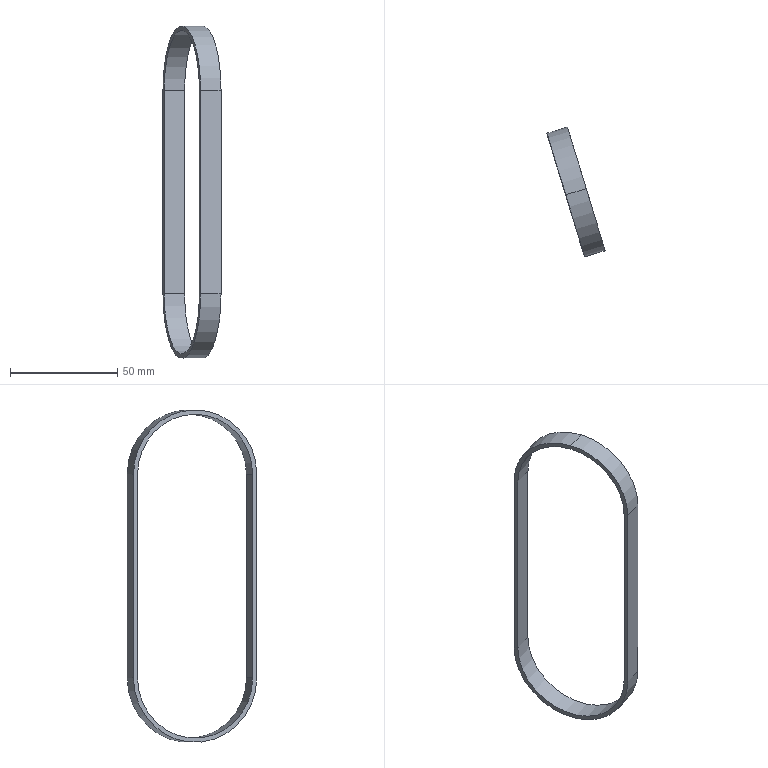Component | SolidWorks | v1_Part1-2112091-1 | 1 solid | 12 faces | box 27.13 x 60.5 x 155.2 mm | volume 7457 mm3 | cylinder 6 | plane 6 | commonest cylinder face diameters 56.2 x3 60.2 x3
build123d program:
from build123d import *

# Parameters (mm, degrees)
EXTRUDE_THIN1_DEPTH = 10


with BuildPart() as part:
    # Sketch1 → Extrude-Thin1 (new body)
    with BuildSketch(Plane.XY):
        with BuildLine():
            Line((95, -30.1), (0, -30.1))
            ThreePointArc((0, -30.1), (-30.1, 0), (0, 30.1))
            Line((0, 30.1), (95, 30.1))
            ThreePointArc((95, 30.1), (125.1, 0), (95, -30.1))
        make_face()
        with BuildLine():
            Line((95, -28.1), (0, -28.1))
            ThreePointArc((0, -28.1), (-28.1, 0), (0, 28.1))
            Line((0, 28.1), (95, 28.1))
            ThreePointArc((95, 28.1), (123.1, 0), (95, -28.1))
        make_face(mode=Mode.SUBTRACT)
    extrude(amount=EXTRUDE_THIN1_DEPTH)


solid = part.part

# Placed as in the assembly
solid = solid.moved(Location((193.934, -227.048, 280.239), (-90, 73.032, -90)))
STEP:
#1=COLOUR_RGB('',0.7922,0.8196,0.9333);
#2=FILL_AREA_STYLE_COLOUR('',#1);
#3=FILL_AREA_STYLE('',(#2));
#4=SURFACE_STYLE_FILL_AREA(#3);
#5=SURFACE_SIDE_STYLE('',(#4));
#6=SURFACE_STYLE_USAGE(.BOTH.,#5);
#7=PRESENTATION_STYLE_ASSIGNMENT((#6));
#8=CARTESIAN_POINT('',(7.689,-7.766,14.773));
#9=VERTEX_POINT('',#8);
#10=CARTESIAN_POINT('',(8.012,-8.824,15.879));
#11=VERTEX_POINT('',#10);
#12=CARTESIAN_POINT('',(8.012,-8.824,14.773));
#13=DIRECTION('',(0.9565,0.2918,0.));
#14=DIRECTION('',(0.,0.,-1.));
#15=AXIS2_PLACEMENT_3D('',#12,#13,#14);
#16=CIRCLE('',#15,1.106);
#17=EDGE_CURVE('',#9,#11,#16,.T.);
#18=ORIENTED_EDGE('',*,*,#17,.T.);
#19=CARTESIAN_POINT('',(7.635,-8.939,15.879));
#20=VERTEX_POINT('',#19);
#21=CARTESIAN_POINT('',(8.012,-8.824,15.879));
#22=DIRECTION('',(-0.9565,-0.2918,-0.));
#23=VECTOR('',#22,39.37);
#24=LINE('',#21,#23);
#25=EDGE_CURVE('',#11,#20,#24,.T.);
#26=ORIENTED_EDGE('',*,*,#25,.T.);
#27=CARTESIAN_POINT('',(7.312,-7.881,14.773));
#28=VERTEX_POINT('',#27);
#29=CARTESIAN_POINT('',(7.635,-8.939,14.773));
#30=DIRECTION('',(0.9565,0.2918,0.));
#31=DIRECTION('',(0.,0.,-1.));
#32=AXIS2_PLACEMENT_3D('',#29,#30,#31);
#33=CIRCLE('',#32,1.106);
#34=EDGE_CURVE('',#28,#20,#33,.T.);
#35=ORIENTED_EDGE('',*,*,#34,.F.);
#36=CARTESIAN_POINT('',(7.689,-7.766,14.773));
#37=DIRECTION('',(-0.9565,-0.2918,-0.));
#38=VECTOR('',#37,39.37);
#39=LINE('',#36,#38);
#40=EDGE_CURVE('',#9,#28,#39,.T.);
#41=ORIENTED_EDGE('',*,*,#40,.F.);
#42=EDGE_LOOP('',(#18,#26,#35,#41));
#43=FACE_OUTER_BOUND('',#42,.T.);
#44=CARTESIAN_POINT('',(8.012,-8.824,14.773));
#45=DIRECTION('',(-0.9565,-0.2918,-0.));
#46=DIRECTION('',(-0.,-0.,1.));
#47=AXIS2_PLACEMENT_3D('',#44,#45,#46);
#48=CYLINDRICAL_SURFACE('',#47,1.106);
#49=ADVANCED_FACE('',(#43),#48,.F.);
#50=CARTESIAN_POINT('',(8.012,-8.824,15.958));
#51=VERTEX_POINT('',#50);
#52=CARTESIAN_POINT('',(8.358,-9.957,14.773));
#53=VERTEX_POINT('',#52);
#54=CARTESIAN_POINT('',(8.012,-8.824,14.773));
#55=DIRECTION('',(0.9565,0.2918,0.));
#56=DIRECTION('',(0.,0.,-1.));
#57=AXIS2_PLACEMENT_3D('',#54,#55,#56);
#58=CIRCLE('',#57,1.185);
#59=EDGE_CURVE('',#51,#53,#58,.T.);
#60=ORIENTED_EDGE('',*,*,#59,.F.);
#61=CARTESIAN_POINT('',(7.635,-8.939,15.958));
#62=VERTEX_POINT('',#61);
#63=CARTESIAN_POINT('',(8.012,-8.824,15.958));
#64=DIRECTION('',(-0.9565,-0.2918,-0.));
#65=VECTOR('',#64,39.37);
#66=LINE('',#63,#65);
#67=EDGE_CURVE('',#51,#62,#66,.T.);
#68=ORIENTED_EDGE('',*,*,#67,.T.);
#69=CARTESIAN_POINT('',(7.981,-10.072,14.773));
#70=VERTEX_POINT('',#69);
#71=CARTESIAN_POINT('',(7.635,-8.939,14.773));
#72=DIRECTION('',(0.9565,0.2918,0.));
#73=DIRECTION('',(0.,0.,-1.));
#74=AXIS2_PLACEMENT_3D('',#71,#72,#73);
#75=CIRCLE('',#74,1.185);
#76=EDGE_CURVE('',#62,#70,#75,.T.);
#77=ORIENTED_EDGE('',*,*,#76,.T.);
#78=CARTESIAN_POINT('',(8.358,-9.957,14.773));
#79=DIRECTION('',(-0.9565,-0.2918,-0.));
#80=VECTOR('',#79,39.37);
#81=LINE('',#78,#80);
#82=EDGE_CURVE('',#53,#70,#81,.T.);
#83=ORIENTED_EDGE('',*,*,#82,.F.);
#84=EDGE_LOOP('',(#60,#68,#77,#83));
#85=FACE_OUTER_BOUND('',#84,.T.);
#86=CARTESIAN_POINT('',(8.012,-8.824,14.773));
#87=DIRECTION('',(-0.9565,-0.2918,-0.));
#88=DIRECTION('',(-0.,-0.,1.));
#89=AXIS2_PLACEMENT_3D('',#86,#87,#88);
#90=CYLINDRICAL_SURFACE('',#89,1.185);
#91=ADVANCED_FACE('',(#85),#90,.T.);
#92=CARTESIAN_POINT('',(8.358,-9.957,11.033));
#93=VERTEX_POINT('',#92);
#94=CARTESIAN_POINT('',(7.666,-7.691,11.033));
#95=VERTEX_POINT('',#94);
#96=CARTESIAN_POINT('',(8.012,-8.824,11.033));
#97=DIRECTION('',(0.9565,0.2918,0.));
#98=DIRECTION('',(0.,0.,-1.));
#99=AXIS2_PLACEMENT_3D('',#96,#97,#98);
#100=CIRCLE('',#99,1.185);
#101=EDGE_CURVE('',#93,#95,#100,.T.);
#102=ORIENTED_EDGE('',*,*,#101,.T.);
#103=CARTESIAN_POINT('',(7.666,-7.691,14.773));
#104=VERTEX_POINT('',#103);
#105=CARTESIAN_POINT('',(7.666,-7.691,14.773));
#106=DIRECTION('',(-0.,-0.,1.));
#107=VECTOR('',#106,39.37);
#108=LINE('',#105,#107);
#109=EDGE_CURVE('',#95,#104,#108,.T.);
#110=ORIENTED_EDGE('',*,*,#109,.T.);
#111=CARTESIAN_POINT('',(8.012,-8.824,14.773));
#112=DIRECTION('',(0.9565,0.2918,0.));
#113=DIRECTION('',(0.,0.,-1.));
#114=AXIS2_PLACEMENT_3D('',#111,#112,#113);
#115=CIRCLE('',#114,1.185);
#116=EDGE_CURVE('',#104,#51,#115,.T.);
#117=ORIENTED_EDGE('',*,*,#116,.T.);
#118=ORIENTED_EDGE('',*,*,#59,.T.);
#119=CARTESIAN_POINT('',(8.358,-9.957,11.033));
#120=DIRECTION('',(0.,0.,-1.));
#121=VECTOR('',#120,39.37);
#122=LINE('',#119,#121);
#123=EDGE_CURVE('',#53,#93,#122,.T.);
#124=ORIENTED_EDGE('',*,*,#123,.T.);
#125=EDGE_LOOP('',(#102,#110,#117,#118,#124));
#126=FACE_OUTER_BOUND('',#125,.T.);
#127=CARTESIAN_POINT('',(7.689,-7.766,11.033));
#128=VERTEX_POINT('',#127);
#129=CARTESIAN_POINT('',(7.689,-7.766,14.773));
#130=DIRECTION('',(-0.,-0.,1.));
#131=VECTOR('',#130,39.37);
#132=LINE('',#129,#131);
#133=EDGE_CURVE('',#128,#9,#132,.T.);
#134=ORIENTED_EDGE('',*,*,#133,.F.);
#135=CARTESIAN_POINT('',(8.335,-9.882,11.033));
#136=VERTEX_POINT('',#135);
#137=CARTESIAN_POINT('',(8.012,-8.824,11.033));
#138=DIRECTION('',(0.9565,0.2918,0.));
#139=DIRECTION('',(0.,0.,-1.));
#140=AXIS2_PLACEMENT_3D('',#137,#138,#139);
#141=CIRCLE('',#140,1.106);
#142=EDGE_CURVE('',#136,#128,#141,.T.);
#143=ORIENTED_EDGE('',*,*,#142,.F.);
#144=CARTESIAN_POINT('',(8.335,-9.882,14.773));
#145=VERTEX_POINT('',#144);
#146=CARTESIAN_POINT('',(8.335,-9.882,11.033));
#147=DIRECTION('',(0.,0.,-1.));
#148=VECTOR('',#147,39.37);
#149=LINE('',#146,#148);
#150=EDGE_CURVE('',#145,#136,#149,.T.);
#151=ORIENTED_EDGE('',*,*,#150,.F.);
#152=CARTESIAN_POINT('',(8.012,-8.824,14.773));
#153=DIRECTION('',(0.9565,0.2918,0.));
#154=DIRECTION('',(0.,0.,-1.));
#155=AXIS2_PLACEMENT_3D('',#152,#153,#154);
#156=CIRCLE('',#155,1.106);
#157=EDGE_CURVE('',#11,#145,#156,.T.);
#158=ORIENTED_EDGE('',*,*,#157,.F.);
#159=ORIENTED_EDGE('',*,*,#17,.F.);
#160=EDGE_LOOP('',(#134,#143,#151,#158,#159));
#161=FACE_BOUND('',#160,.T.);
#162=CARTESIAN_POINT('',(8.012,-8.824,11.033));
#163=DIRECTION('',(0.9565,0.2918,0.));
#164=DIRECTION('',(0.,0.,-1.));
#165=AXIS2_PLACEMENT_3D('',#162,#163,#164);
#166=PLANE('',#165);
#167=ADVANCED_FACE('',(#126,#161),#166,.T.);
#168=CARTESIAN_POINT('',(7.981,-10.072,11.033));
#169=VERTEX_POINT('',#168);
#170=CARTESIAN_POINT('',(7.289,-7.805,11.033));
#171=VERTEX_POINT('',#170);
#172=CARTESIAN_POINT('',(7.635,-8.939,11.033));
#173=DIRECTION('',(0.9565,0.2918,0.));
#174=DIRECTION('',(0.,0.,-1.));
#175=AXIS2_PLACEMENT_3D('',#172,#173,#174);
#176=CIRCLE('',#175,1.185);
#177=EDGE_CURVE('',#169,#171,#176,.T.);
#178=ORIENTED_EDGE('',*,*,#177,.F.);
#179=CARTESIAN_POINT('',(7.981,-10.072,11.033));
#180=DIRECTION('',(0.,0.,-1.));
#181=VECTOR('',#180,39.37);
#182=LINE('',#179,#181);
#183=EDGE_CURVE('',#70,#169,#182,.T.);
#184=ORIENTED_EDGE('',*,*,#183,.F.);
#185=ORIENTED_EDGE('',*,*,#76,.F.);
#186=CARTESIAN_POINT('',(7.289,-7.805,14.773));
#187=VERTEX_POINT('',#186);
#188=CARTESIAN_POINT('',(7.635,-8.939,14.773));
#189=DIRECTION('',(0.9565,0.2918,0.));
#190=DIRECTION('',(0.,0.,-1.));
#191=AXIS2_PLACEMENT_3D('',#188,#189,#190);
#192=CIRCLE('',#191,1.185);
#193=EDGE_CURVE('',#187,#62,#192,.T.);
#194=ORIENTED_EDGE('',*,*,#193,.F.);
#195=CARTESIAN_POINT('',(7.289,-7.805,14.773));
#196=DIRECTION('',(-0.,-0.,1.));
#197=VECTOR('',#196,39.37);
#198=LINE('',#195,#197);
#199=EDGE_CURVE('',#171,#187,#198,.T.);
#200=ORIENTED_EDGE('',*,*,#199,.F.);
#201=EDGE_LOOP('',(#178,#184,#185,#194,#200));
#202=FACE_OUTER_BOUND('',#201,.T.);
#203=CARTESIAN_POINT('',(7.958,-9.997,11.033));
#204=VERTEX_POINT('',#203);
#205=CARTESIAN_POINT('',(7.312,-7.881,11.033));
#206=VERTEX_POINT('',#205);
#207=CARTESIAN_POINT('',(7.635,-8.939,11.033));
#208=DIRECTION('',(0.9565,0.2918,0.));
#209=DIRECTION('',(0.,0.,-1.));
#210=AXIS2_PLACEMENT_3D('',#207,#208,#209);
#211=CIRCLE('',#210,1.106);
#212=EDGE_CURVE('',#204,#206,#211,.T.);
#213=ORIENTED_EDGE('',*,*,#212,.T.);
#214=CARTESIAN_POINT('',(7.312,-7.881,14.773));
#215=DIRECTION('',(-0.,-0.,1.));
#216=VECTOR('',#215,39.37);
#217=LINE('',#214,#216);
#218=EDGE_CURVE('',#206,#28,#217,.T.);
#219=ORIENTED_EDGE('',*,*,#218,.T.);
#220=ORIENTED_EDGE('',*,*,#34,.T.);
#221=CARTESIAN_POINT('',(7.958,-9.997,14.773));
#222=VERTEX_POINT('',#221);
#223=CARTESIAN_POINT('',(7.635,-8.939,14.773));
#224=DIRECTION('',(0.9565,0.2918,0.));
#225=DIRECTION('',(0.,0.,-1.));
#226=AXIS2_PLACEMENT_3D('',#223,#224,#225);
#227=CIRCLE('',#226,1.106);
#228=EDGE_CURVE('',#20,#222,#227,.T.);
#229=ORIENTED_EDGE('',*,*,#228,.T.);
#230=CARTESIAN_POINT('',(7.958,-9.997,11.033));
#231=DIRECTION('',(0.,0.,-1.));
#232=VECTOR('',#231,39.37);
#233=LINE('',#230,#232);
#234=EDGE_CURVE('',#222,#204,#233,.T.);
#235=ORIENTED_EDGE('',*,*,#234,.T.);
#236=EDGE_LOOP('',(#213,#219,#220,#229,#235));
#237=FACE_BOUND('',#236,.T.);
#238=CARTESIAN_POINT('',(7.635,-8.939,11.033));
#239=DIRECTION('',(0.9565,0.2918,0.));
#240=DIRECTION('',(0.,0.,-1.));
#241=AXIS2_PLACEMENT_3D('',#238,#239,#240);
#242=PLANE('',#241);
#243=ADVANCED_FACE('',(#202,#237),#242,.F.);
#244=ORIENTED_EDGE('',*,*,#177,.T.);
#245=CARTESIAN_POINT('',(7.666,-7.691,11.033));
#246=DIRECTION('',(-0.9565,-0.2918,-0.));
#247=VECTOR('',#246,39.37);
#248=LINE('',#245,#247);
#249=EDGE_CURVE('',#95,#171,#248,.T.);
#250=ORIENTED_EDGE('',*,*,#249,.F.);
#251=ORIENTED_EDGE('',*,*,#101,.F.);
#252=CARTESIAN_POINT('',(8.358,-9.957,11.033));
#253=DIRECTION('',(-0.9565,-0.2918,-0.));
#254=VECTOR('',#253,39.37);
#255=LINE('',#252,#254);
#256=EDGE_CURVE('',#93,#169,#255,.T.);
#257=ORIENTED_EDGE('',*,*,#256,.T.);
#258=EDGE_LOOP('',(#244,#250,#251,#257));
#259=FACE_OUTER_BOUND('',#258,.T.);
#260=CARTESIAN_POINT('',(8.012,-8.824,11.033));
#261=DIRECTION('',(-0.9565,-0.2918,-0.));
#262=DIRECTION('',(-0.,-0.,1.));
#263=AXIS2_PLACEMENT_3D('',#260,#261,#262);
#264=CYLINDRICAL_SURFACE('',#263,1.185);
#265=ADVANCED_FACE('',(#259),#264,.T.);
#266=ORIENTED_EDGE('',*,*,#199,.T.);
#267=CARTESIAN_POINT('',(7.666,-7.691,14.773));
#268=DIRECTION('',(-0.9565,-0.2918,-0.));
#269=VECTOR('',#268,39.37);
#270=LINE('',#267,#269);
#271=EDGE_CURVE('',#104,#187,#270,.T.);
#272=ORIENTED_EDGE('',*,*,#271,.F.);
#273=ORIENTED_EDGE('',*,*,#109,.F.);
#274=ORIENTED_EDGE('',*,*,#249,.T.);
#275=EDGE_LOOP('',(#266,#272,#273,#274));
#276=FACE_OUTER_BOUND('',#275,.T.);
#277=CARTESIAN_POINT('',(7.666,-7.691,14.773));
#278=DIRECTION('',(0.2918,-0.9565,-0.));
#279=DIRECTION('',(-0.9565,-0.2918,-0.));
#280=AXIS2_PLACEMENT_3D('',#277,#278,#279);
#281=PLANE('',#280);
#282=ADVANCED_FACE('',(#276),#281,.F.);
#283=ORIENTED_EDGE('',*,*,#67,.F.);
#284=ORIENTED_EDGE('',*,*,#116,.F.);
#285=ORIENTED_EDGE('',*,*,#271,.T.);
#286=ORIENTED_EDGE('',*,*,#193,.T.);
#287=EDGE_LOOP('',(#283,#284,#285,#286));
#288=FACE_OUTER_BOUND('',#287,.T.);
#289=CARTESIAN_POINT('',(8.012,-8.824,14.773));
#290=DIRECTION('',(-0.9565,-0.2918,-0.));
#291=DIRECTION('',(-0.,-0.,1.));
#292=AXIS2_PLACEMENT_3D('',#289,#290,#291);
#293=CYLINDRICAL_SURFACE('',#292,1.185);
#294=ADVANCED_FACE('',(#288),#293,.T.);
#295=ORIENTED_EDGE('',*,*,#183,.T.);
#296=ORIENTED_EDGE('',*,*,#256,.F.);
#297=ORIENTED_EDGE('',*,*,#123,.F.);
#298=ORIENTED_EDGE('',*,*,#82,.T.);
#299=EDGE_LOOP('',(#295,#296,#297,#298));
#300=FACE_OUTER_BOUND('',#299,.T.);
#301=CARTESIAN_POINT('',(8.358,-9.957,11.033));
#302=DIRECTION('',(-0.2918,0.9565,0.));
#303=DIRECTION('',(0.9565,0.2918,0.));
#304=AXIS2_PLACEMENT_3D('',#301,#302,#303);
#305=PLANE('',#304);
#306=ADVANCED_FACE('',(#300),#305,.F.);
#307=ORIENTED_EDGE('',*,*,#212,.F.);
#308=CARTESIAN_POINT('',(8.335,-9.882,11.033));
#309=DIRECTION('',(-0.9565,-0.2918,-0.));
#310=VECTOR('',#309,39.37);
#311=LINE('',#308,#310);
#312=EDGE_CURVE('',#136,#204,#311,.T.);
#313=ORIENTED_EDGE('',*,*,#312,.F.);
#314=ORIENTED_EDGE('',*,*,#142,.T.);
#315=CARTESIAN_POINT('',(7.689,-7.766,11.033));
#316=DIRECTION('',(-0.9565,-0.2918,-0.));
#317=VECTOR('',#316,39.37);
#318=LINE('',#315,#317);
#319=EDGE_CURVE('',#128,#206,#318,.T.);
#320=ORIENTED_EDGE('',*,*,#319,.T.);
#321=EDGE_LOOP('',(#307,#313,#314,#320));
#322=FACE_OUTER_BOUND('',#321,.T.);
#323=CARTESIAN_POINT('',(8.012,-8.824,11.033));
#324=DIRECTION('',(-0.9565,-0.2918,-0.));
#325=DIRECTION('',(-0.,-0.,1.));
#326=AXIS2_PLACEMENT_3D('',#323,#324,#325);
#327=CYLINDRICAL_SURFACE('',#326,1.106);
#328=ADVANCED_FACE('',(#322),#327,.F.);
#329=ORIENTED_EDGE('',*,*,#218,.F.);
#330=ORIENTED_EDGE('',*,*,#319,.F.);
#331=ORIENTED_EDGE('',*,*,#133,.T.);
#332=ORIENTED_EDGE('',*,*,#40,.T.);
#333=EDGE_LOOP('',(#329,#330,#331,#332));
#334=FACE_OUTER_BOUND('',#333,.T.);
#335=CARTESIAN_POINT('',(7.689,-7.766,14.773));
#336=DIRECTION('',(0.2918,-0.9565,-0.));
#337=DIRECTION('',(-0.9565,-0.2918,-0.));
#338=AXIS2_PLACEMENT_3D('',#335,#336,#337);
#339=PLANE('',#338);
#340=ADVANCED_FACE('',(#334),#339,.T.);
#341=ORIENTED_EDGE('',*,*,#25,.F.);
#342=ORIENTED_EDGE('',*,*,#157,.T.);
#343=CARTESIAN_POINT('',(8.335,-9.882,14.773));
#344=DIRECTION('',(-0.9565,-0.2918,-0.));
#345=VECTOR('',#344,39.37);
#346=LINE('',#343,#345);
#347=EDGE_CURVE('',#145,#222,#346,.T.);
#348=ORIENTED_EDGE('',*,*,#347,.T.);
#349=ORIENTED_EDGE('',*,*,#228,.F.);
#350=EDGE_LOOP('',(#341,#342,#348,#349));
#351=FACE_OUTER_BOUND('',#350,.T.);
#352=CARTESIAN_POINT('',(8.012,-8.824,14.773));
#353=DIRECTION('',(-0.9565,-0.2918,-0.));
#354=DIRECTION('',(-0.,-0.,1.));
#355=AXIS2_PLACEMENT_3D('',#352,#353,#354);
#356=CYLINDRICAL_SURFACE('',#355,1.106);
#357=ADVANCED_FACE('',(#351),#356,.F.);
#358=ORIENTED_EDGE('',*,*,#234,.F.);
#359=ORIENTED_EDGE('',*,*,#347,.F.);
#360=ORIENTED_EDGE('',*,*,#150,.T.);
#361=ORIENTED_EDGE('',*,*,#312,.T.);
#362=EDGE_LOOP('',(#358,#359,#360,#361));
#363=FACE_OUTER_BOUND('',#362,.T.);
#364=CARTESIAN_POINT('',(8.335,-9.882,11.033));
#365=DIRECTION('',(-0.2918,0.9565,0.));
#366=DIRECTION('',(0.9565,0.2918,0.));
#367=AXIS2_PLACEMENT_3D('',#364,#365,#366);
#368=PLANE('',#367);
#369=ADVANCED_FACE('',(#363),#368,.T.);
#370=CLOSED_SHELL('',(#49,#91,#167,#243,#265,#282,#294,#306,#328,#340,#357,#369));
#371=MANIFOLD_SOLID_BREP('',#370);
#372=STYLED_ITEM('',(#7),#371);
#373=PRESENTATION_LAYER_ASSIGNMENT('','',(#372));
#374=(LENGTH_UNIT()NAMED_UNIT(*)SI_UNIT($,.METRE.));
#375=LENGTH_MEASURE_WITH_UNIT(LENGTH_MEASURE(0.0254),#374);
#376=DIMENSIONAL_EXPONENTS(1.,0.,0.,0.,0.,0.,0.);
#377=(CONVERSION_BASED_UNIT('',#375)LENGTH_UNIT()NAMED_UNIT(#376));
#378=UNCERTAINTY_MEASURE_WITH_UNIT(LENGTH_MEASURE(0.00001),#377,'','');
#379=(NAMED_UNIT(*)PLANE_ANGLE_UNIT()SI_UNIT($,.RADIAN.));
#380=(NAMED_UNIT(*)SI_UNIT($,.STERADIAN.)SOLID_ANGLE_UNIT());
#381=(GEOMETRIC_REPRESENTATION_CONTEXT(3)GLOBAL_UNCERTAINTY_ASSIGNED_CONTEXT((#378))GLOBAL_UNIT_ASSIGNED_CONTEXT((#377,#379,#380))REPRESENTATION_CONTEXT('',''));
#382=MECHANICAL_DESIGN_GEOMETRIC_PRESENTATION_REPRESENTATION('',(#372),#381);
#383=CARTESIAN_POINT('',(0.,0.,0.));
#384=DIRECTION('',(0.,0.,1.));
#385=DIRECTION('',(1.,0.,0.));
#386=AXIS2_PLACEMENT_3D('',#383,#384,#385);
#387=(LENGTH_UNIT()NAMED_UNIT(*)SI_UNIT($,.METRE.));
#388=LENGTH_MEASURE_WITH_UNIT(LENGTH_MEASURE(0.0254),#387);
#389=DIMENSIONAL_EXPONENTS(1.,0.,0.,0.,0.,0.,0.);
#390=(CONVERSION_BASED_UNIT('',#388)LENGTH_UNIT()NAMED_UNIT(#389));
#391=UNCERTAINTY_MEASURE_WITH_UNIT(LENGTH_MEASURE(0.00001),#390,'','');
#392=(NAMED_UNIT(*)PLANE_ANGLE_UNIT()SI_UNIT($,.RADIAN.));
#393=(NAMED_UNIT(*)SI_UNIT($,.STERADIAN.)SOLID_ANGLE_UNIT());
#394=(GEOMETRIC_REPRESENTATION_CONTEXT(3)GLOBAL_UNCERTAINTY_ASSIGNED_CONTEXT((#391))GLOBAL_UNIT_ASSIGNED_CONTEXT((#390,#392,#393))REPRESENTATION_CONTEXT('',''));
#395=ADVANCED_BREP_SHAPE_REPRESENTATION('',(#371,#386),#394);